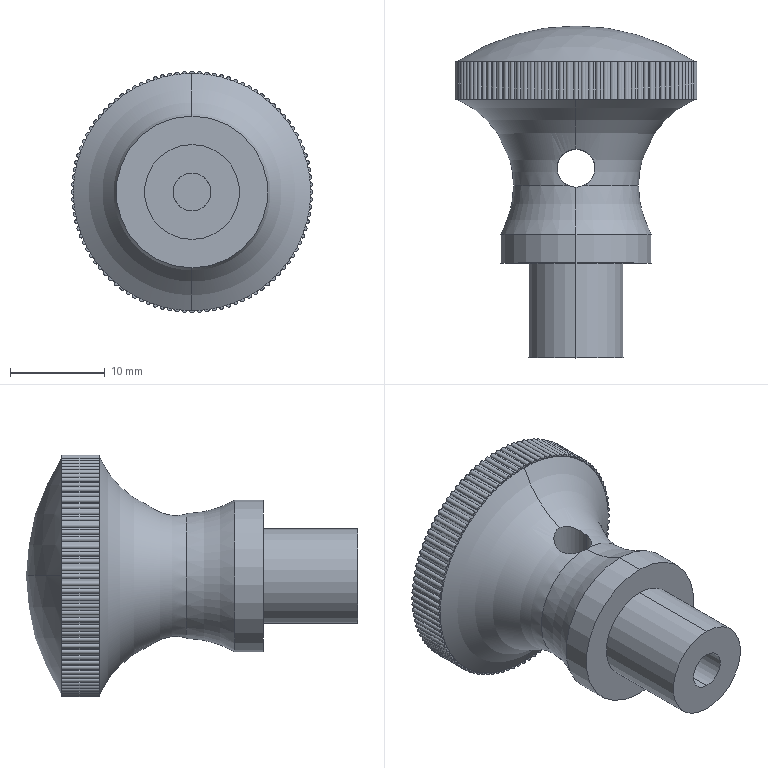Component | SolidWorks | UpperHousingAssembly-1_VentCap-1 | 1 solid | 474 faces | box 25.5 x 35 x 25.5 mm | volume 6761 mm3 | cylinder 265 | plane 203 | torus 4 | sphere 2 | commonest cylinder face diameters 0.5 x153 25 x100 4 x8 10 x2 16 x2
build123d program:
from build123d import *

# Parameters (mm, degrees)
SKETCH8_R           = 2
CUT_EXTRUDE4_DEPTH  = 10
SKETCH9_R           = 0.25
BOSS_EXTRUDE2_DEPTH = 4
CIRPATTERN3_COUNT   = 100
SKETCH10_R          = 2
CUT_EXTRUDE6_DEPTH  = 22


with BuildPart() as part:
    # Sketch7 → Revolve3 (revolve)
    with BuildSketch(Plane.XY, mode=Mode.PRIVATE) as revolve3_sk:
        with BuildLine():
            Line((0, 35), (0, 0))
            Line((0, 0), (5, 0))
            Line((5, 0), (5, 10))
            Line((5, 10), (8, 10))
            Line((8, 10), (8, 13))
            ThreePointArc((8, 13), (7.049, 21.138), (12.5, 27.255))
            Line((12.5, 27.255), (12.5, 31.255))
            ThreePointArc((12.5, 31.255), (6.524, 34.044), (0, 35))
        make_face()
    revolve(revolve3_sk.sketch.rotate(Axis((0, 0, 0), (0, 1, 0)), 90), axis=Axis((0, 0, 0), (0, 1, 0)))

    # Sketch8 → Cut-Extrude4 (cut, symmetric)
    with BuildSketch(Plane.XY):
        with Locations(Location((0, 20, 0), (0, 0, 270))):
            Circle(SKETCH8_R)
    extrude(amount=CUT_EXTRUDE4_DEPTH, both=True, mode=Mode.SUBTRACT)

    # Sketch9 → Boss-Extrude2 (add)
    with BuildSketch(Plane(origin=(0, 27.255, 0), x_dir=(-1, 0, 0), z_dir=(0, -1, 0))):
        with Locations((-12.5, 0)):
            Circle(SKETCH9_R)
    boss_extrude2 = extrude(amount=-BOSS_EXTRUDE2_DEPTH)

    # CirPattern3: Boss-Extrude2 ×100 about axis
    cirpattern3_axis = Axis((0, 0, 0), (0, 1, 0))
    for i in range(1, CIRPATTERN3_COUNT):
        add(boss_extrude2.rotate(cirpattern3_axis, i * 360 / CIRPATTERN3_COUNT))

    # Sketch10 → Cut-Extrude6 (cut)
    with BuildSketch(Plane.XZ):
        with Locations(Location((0, 0, 0), (0, 0, 270))):
            Circle(SKETCH10_R)
    extrude(amount=-CUT_EXTRUDE6_DEPTH, mode=Mode.SUBTRACT)


solid = part.part

# Placed as in the assembly
solid = solid.moved(Location((895.83, 1537.591, 1632.217), (0, 0, 0)))